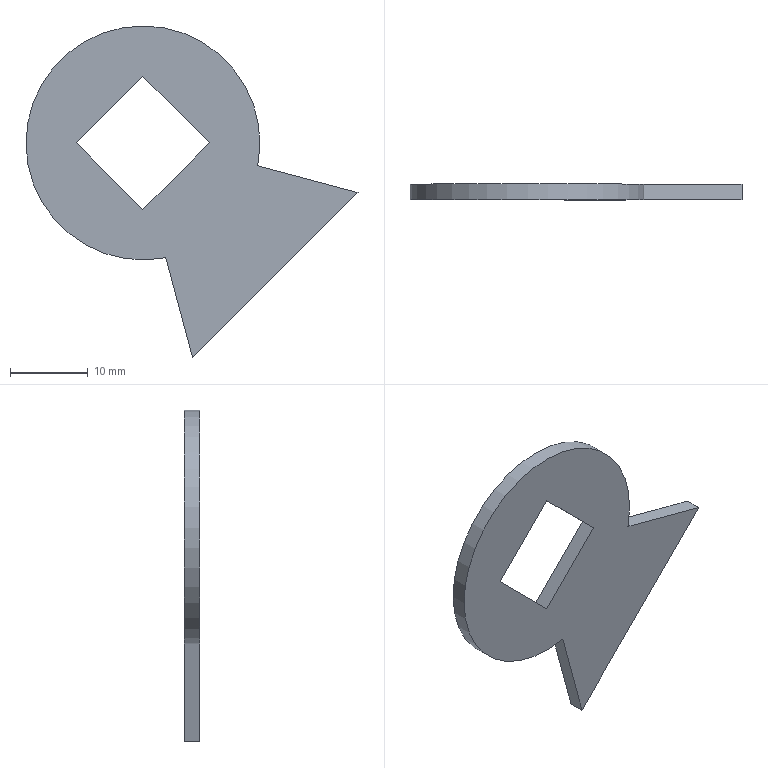Component | NX | LIMIT_PLATE | 1 solid | 10 faces | box 42.58 x 2 x 42.58 mm | volume 1607 mm3 | plane 9 | cylinder 1 | commonest cylinder face diameters 30 x1
STEP:
#1=CARTESIAN_POINT('',(0.,0.,0.));
#2=DIRECTION('',(0.,0.,1.));
#3=DIRECTION('',(1.,0.,0.));
#4=AXIS2_PLACEMENT_3D('',#1,#2,#3);
#5=CARTESIAN_POINT('',(-0.,-95.,-35.485));
#6=VERTEX_POINT('',#5);
#7=CARTESIAN_POINT('',(-8.485,-95.,-27.));
#8=VERTEX_POINT('',#7);
#9=CARTESIAN_POINT('',(-0.,-95.,-35.485));
#10=DIRECTION('',(-0.7071,0.,0.7071));
#11=VECTOR('',#10,1.);
#12=LINE('',#9,#11);
#13=CARTESIAN_POINT('',(-0.,-97.,-35.485));
#14=DIRECTION('',(-0.7071,0.,-0.7071));
#15=DIRECTION('',(0.7071,0.,-0.7071));
#16=AXIS2_PLACEMENT_3D('',#13,#14,#15);
#17=PLANE('',#16);
#18=CARTESIAN_POINT('',(0.,-2.));
#19=DIRECTION('',(-1.,0.));
#20=VECTOR('',#19,1.);
#21=LINE('',#18,#20);
#22=(GEOMETRIC_REPRESENTATION_CONTEXT(2)PARAMETRIC_REPRESENTATION_CONTEXT()REPRESENTATION_CONTEXT('',''));
#23=DEFINITIONAL_REPRESENTATION('',(#21),#22);
#24=PCURVE('',#17,#23);
#25=CARTESIAN_POINT('',(0.,-95.,-27.));
#26=DIRECTION('',(0.,1.,0.));
#27=DIRECTION('',(-0.7071,0.,-0.7071));
#28=AXIS2_PLACEMENT_3D('',#25,#26,#27);
#29=PLANE('',#28);
#30=CARTESIAN_POINT('',(6.,-6.));
#31=DIRECTION('',(0.,1.));
#32=VECTOR('',#31,1.);
#33=LINE('',#30,#32);
#34=(GEOMETRIC_REPRESENTATION_CONTEXT(2)PARAMETRIC_REPRESENTATION_CONTEXT()REPRESENTATION_CONTEXT('',''));
#35=DEFINITIONAL_REPRESENTATION('',(#33),#34);
#36=PCURVE('',#29,#35);
#37=SURFACE_CURVE('',#12,(#24,#36),.PCURVE_S1.);
#38=EDGE_CURVE('',#6,#8,#37,.T.);
#39=ORIENTED_EDGE('',*,*,#38,.T.);
#40=CARTESIAN_POINT('',(-8.485,-97.,-27.));
#41=VERTEX_POINT('',#40);
#42=CARTESIAN_POINT('',(-8.485,-97.,-27.));
#43=DIRECTION('',(0.,1.,0.));
#44=VECTOR('',#43,1.);
#45=LINE('',#42,#44);
#46=CARTESIAN_POINT('',(-12.,0.));
#47=DIRECTION('',(0.,-1.));
#48=VECTOR('',#47,1.);
#49=LINE('',#46,#48);
#50=(GEOMETRIC_REPRESENTATION_CONTEXT(2)PARAMETRIC_REPRESENTATION_CONTEXT()REPRESENTATION_CONTEXT('',''));
#51=DEFINITIONAL_REPRESENTATION('',(#49),#50);
#52=PCURVE('',#17,#51);
#53=CARTESIAN_POINT('',(-8.485,-97.,-27.));
#54=DIRECTION('',(-0.7071,0.,0.7071));
#55=DIRECTION('',(-0.7071,0.,-0.7071));
#56=AXIS2_PLACEMENT_3D('',#53,#54,#55);
#57=PLANE('',#56);
#58=CARTESIAN_POINT('',(0.,0.));
#59=DIRECTION('',(0.,-1.));
#60=VECTOR('',#59,1.);
#61=LINE('',#58,#60);
#62=(GEOMETRIC_REPRESENTATION_CONTEXT(2)PARAMETRIC_REPRESENTATION_CONTEXT()REPRESENTATION_CONTEXT('',''));
#63=DEFINITIONAL_REPRESENTATION('',(#61),#62);
#64=PCURVE('',#57,#63);
#65=SURFACE_CURVE('',#45,(#52,#64),.PCURVE_S1.);
#66=EDGE_CURVE('',#41,#8,#65,.T.);
#67=ORIENTED_EDGE('',*,*,#66,.F.);
#68=CARTESIAN_POINT('',(-0.,-97.,-35.485));
#69=VERTEX_POINT('',#68);
#70=CARTESIAN_POINT('',(-0.,-97.,-35.485));
#71=DIRECTION('',(-0.7071,0.,0.7071));
#72=VECTOR('',#71,1.);
#73=LINE('',#70,#72);
#74=CARTESIAN_POINT('',(0.,0.));
#75=DIRECTION('',(-1.,0.));
#76=VECTOR('',#75,1.);
#77=LINE('',#74,#76);
#78=(GEOMETRIC_REPRESENTATION_CONTEXT(2)PARAMETRIC_REPRESENTATION_CONTEXT()REPRESENTATION_CONTEXT('',''));
#79=DEFINITIONAL_REPRESENTATION('',(#77),#78);
#80=PCURVE('',#17,#79);
#81=CARTESIAN_POINT('',(0.,-97.,-27.));
#82=DIRECTION('',(0.,1.,0.));
#83=DIRECTION('',(-0.7071,0.,-0.7071));
#84=AXIS2_PLACEMENT_3D('',#81,#82,#83);
#85=PLANE('',#84);
#86=CARTESIAN_POINT('',(6.,-6.));
#87=DIRECTION('',(0.,1.));
#88=VECTOR('',#87,1.);
#89=LINE('',#86,#88);
#90=(GEOMETRIC_REPRESENTATION_CONTEXT(2)PARAMETRIC_REPRESENTATION_CONTEXT()REPRESENTATION_CONTEXT('',''));
#91=DEFINITIONAL_REPRESENTATION('',(#89),#90);
#92=PCURVE('',#85,#91);
#93=SURFACE_CURVE('',#73,(#80,#92),.PCURVE_S1.);
#94=EDGE_CURVE('',#69,#41,#93,.T.);
#95=ORIENTED_EDGE('',*,*,#94,.F.);
#96=CARTESIAN_POINT('',(-0.,-97.,-35.485));
#97=DIRECTION('',(0.,1.,0.));
#98=VECTOR('',#97,1.);
#99=LINE('',#96,#98);
#100=CARTESIAN_POINT('',(0.,0.));
#101=DIRECTION('',(0.,-1.));
#102=VECTOR('',#101,1.);
#103=LINE('',#100,#102);
#104=(GEOMETRIC_REPRESENTATION_CONTEXT(2)PARAMETRIC_REPRESENTATION_CONTEXT()REPRESENTATION_CONTEXT('',''));
#105=DEFINITIONAL_REPRESENTATION('',(#103),#104);
#106=PCURVE('',#17,#105);
#107=CARTESIAN_POINT('',(8.485,-97.,-27.));
#108=DIRECTION('',(0.7071,0.,-0.7071));
#109=DIRECTION('',(0.7071,0.,0.7071));
#110=AXIS2_PLACEMENT_3D('',#107,#108,#109);
#111=PLANE('',#110);
#112=CARTESIAN_POINT('',(-12.,0.));
#113=DIRECTION('',(0.,-1.));
#114=VECTOR('',#113,1.);
#115=LINE('',#112,#114);
#116=(GEOMETRIC_REPRESENTATION_CONTEXT(2)PARAMETRIC_REPRESENTATION_CONTEXT()REPRESENTATION_CONTEXT('',''));
#117=DEFINITIONAL_REPRESENTATION('',(#115),#116);
#118=PCURVE('',#111,#117);
#119=SURFACE_CURVE('',#99,(#106,#118),.PCURVE_S1.);
#120=EDGE_CURVE('',#69,#6,#119,.T.);
#121=ORIENTED_EDGE('',*,*,#120,.T.);
#122=EDGE_LOOP('',(#39,#67,#95,#121));
#123=FACE_BOUND('',#122,.T.);
#124=ADVANCED_FACE('',(#123),#17,.F.);
#125=CARTESIAN_POINT('',(8.485,-95.,-27.));
#126=VERTEX_POINT('',#125);
#127=CARTESIAN_POINT('',(8.485,-95.,-27.));
#128=DIRECTION('',(-0.7071,0.,-0.7071));
#129=VECTOR('',#128,1.);
#130=LINE('',#127,#129);
#131=CARTESIAN_POINT('',(0.,-2.));
#132=DIRECTION('',(-1.,0.));
#133=VECTOR('',#132,1.);
#134=LINE('',#131,#133);
#135=(GEOMETRIC_REPRESENTATION_CONTEXT(2)PARAMETRIC_REPRESENTATION_CONTEXT()REPRESENTATION_CONTEXT('',''));
#136=DEFINITIONAL_REPRESENTATION('',(#134),#135);
#137=PCURVE('',#111,#136);
#138=CARTESIAN_POINT('',(-6.,-6.));
#139=DIRECTION('',(1.,0.));
#140=VECTOR('',#139,1.);
#141=LINE('',#138,#140);
#142=(GEOMETRIC_REPRESENTATION_CONTEXT(2)PARAMETRIC_REPRESENTATION_CONTEXT()REPRESENTATION_CONTEXT('',''));
#143=DEFINITIONAL_REPRESENTATION('',(#141),#142);
#144=PCURVE('',#29,#143);
#145=SURFACE_CURVE('',#130,(#137,#144),.PCURVE_S1.);
#146=EDGE_CURVE('',#126,#6,#145,.T.);
#147=ORIENTED_EDGE('',*,*,#146,.T.);
#148=ORIENTED_EDGE('',*,*,#120,.F.);
#149=CARTESIAN_POINT('',(8.485,-97.,-27.));
#150=VERTEX_POINT('',#149);
#151=CARTESIAN_POINT('',(8.485,-97.,-27.));
#152=DIRECTION('',(-0.7071,0.,-0.7071));
#153=VECTOR('',#152,1.);
#154=LINE('',#151,#153);
#155=CARTESIAN_POINT('',(0.,0.));
#156=DIRECTION('',(-1.,0.));
#157=VECTOR('',#156,1.);
#158=LINE('',#155,#157);
#159=(GEOMETRIC_REPRESENTATION_CONTEXT(2)PARAMETRIC_REPRESENTATION_CONTEXT()REPRESENTATION_CONTEXT('',''));
#160=DEFINITIONAL_REPRESENTATION('',(#158),#159);
#161=PCURVE('',#111,#160);
#162=CARTESIAN_POINT('',(-6.,-6.));
#163=DIRECTION('',(1.,0.));
#164=VECTOR('',#163,1.);
#165=LINE('',#162,#164);
#166=(GEOMETRIC_REPRESENTATION_CONTEXT(2)PARAMETRIC_REPRESENTATION_CONTEXT()REPRESENTATION_CONTEXT('',''));
#167=DEFINITIONAL_REPRESENTATION('',(#165),#166);
#168=PCURVE('',#85,#167);
#169=SURFACE_CURVE('',#154,(#161,#168),.PCURVE_S1.);
#170=EDGE_CURVE('',#150,#69,#169,.T.);
#171=ORIENTED_EDGE('',*,*,#170,.F.);
#172=CARTESIAN_POINT('',(8.485,-97.,-27.));
#173=DIRECTION('',(0.,1.,0.));
#174=VECTOR('',#173,1.);
#175=LINE('',#172,#174);
#176=CARTESIAN_POINT('',(0.,0.));
#177=DIRECTION('',(0.,-1.));
#178=VECTOR('',#177,1.);
#179=LINE('',#176,#178);
#180=(GEOMETRIC_REPRESENTATION_CONTEXT(2)PARAMETRIC_REPRESENTATION_CONTEXT()REPRESENTATION_CONTEXT('',''));
#181=DEFINITIONAL_REPRESENTATION('',(#179),#180);
#182=PCURVE('',#111,#181);
#183=CARTESIAN_POINT('',(0.,-97.,-18.515));
#184=DIRECTION('',(0.7071,0.,0.7071));
#185=DIRECTION('',(-0.7071,0.,0.7071));
#186=AXIS2_PLACEMENT_3D('',#183,#184,#185);
#187=PLANE('',#186);
#188=CARTESIAN_POINT('',(-12.,0.));
#189=DIRECTION('',(0.,-1.));
#190=VECTOR('',#189,1.);
#191=LINE('',#188,#190);
#192=(GEOMETRIC_REPRESENTATION_CONTEXT(2)PARAMETRIC_REPRESENTATION_CONTEXT()REPRESENTATION_CONTEXT('',''));
#193=DEFINITIONAL_REPRESENTATION('',(#191),#192);
#194=PCURVE('',#187,#193);
#195=SURFACE_CURVE('',#175,(#182,#194),.PCURVE_S1.);
#196=EDGE_CURVE('',#150,#126,#195,.T.);
#197=ORIENTED_EDGE('',*,*,#196,.T.);
#198=EDGE_LOOP('',(#147,#148,#171,#197));
#199=FACE_BOUND('',#198,.T.);
#200=ADVANCED_FACE('',(#199),#111,.F.);
#201=CARTESIAN_POINT('',(0.,-95.,-18.515));
#202=VERTEX_POINT('',#201);
#203=CARTESIAN_POINT('',(0.,-95.,-18.515));
#204=DIRECTION('',(0.7071,0.,-0.7071));
#205=VECTOR('',#204,1.);
#206=LINE('',#203,#205);
#207=CARTESIAN_POINT('',(0.,-2.));
#208=DIRECTION('',(-1.,0.));
#209=VECTOR('',#208,1.);
#210=LINE('',#207,#209);
#211=(GEOMETRIC_REPRESENTATION_CONTEXT(2)PARAMETRIC_REPRESENTATION_CONTEXT()REPRESENTATION_CONTEXT('',''));
#212=DEFINITIONAL_REPRESENTATION('',(#210),#211);
#213=PCURVE('',#187,#212);
#214=CARTESIAN_POINT('',(-6.,6.));
#215=DIRECTION('',(0.,-1.));
#216=VECTOR('',#215,1.);
#217=LINE('',#214,#216);
#218=(GEOMETRIC_REPRESENTATION_CONTEXT(2)PARAMETRIC_REPRESENTATION_CONTEXT()REPRESENTATION_CONTEXT('',''));
#219=DEFINITIONAL_REPRESENTATION('',(#217),#218);
#220=PCURVE('',#29,#219);
#221=SURFACE_CURVE('',#206,(#213,#220),.PCURVE_S1.);
#222=EDGE_CURVE('',#202,#126,#221,.T.);
#223=ORIENTED_EDGE('',*,*,#222,.T.);
#224=ORIENTED_EDGE('',*,*,#196,.F.);
#225=CARTESIAN_POINT('',(0.,-97.,-18.515));
#226=VERTEX_POINT('',#225);
#227=CARTESIAN_POINT('',(0.,-97.,-18.515));
#228=DIRECTION('',(0.7071,0.,-0.7071));
#229=VECTOR('',#228,1.);
#230=LINE('',#227,#229);
#231=CARTESIAN_POINT('',(0.,0.));
#232=DIRECTION('',(-1.,0.));
#233=VECTOR('',#232,1.);
#234=LINE('',#231,#233);
#235=(GEOMETRIC_REPRESENTATION_CONTEXT(2)PARAMETRIC_REPRESENTATION_CONTEXT()REPRESENTATION_CONTEXT('',''));
#236=DEFINITIONAL_REPRESENTATION('',(#234),#235);
#237=PCURVE('',#187,#236);
#238=CARTESIAN_POINT('',(-6.,6.));
#239=DIRECTION('',(0.,-1.));
#240=VECTOR('',#239,1.);
#241=LINE('',#238,#240);
#242=(GEOMETRIC_REPRESENTATION_CONTEXT(2)PARAMETRIC_REPRESENTATION_CONTEXT()REPRESENTATION_CONTEXT('',''));
#243=DEFINITIONAL_REPRESENTATION('',(#241),#242);
#244=PCURVE('',#85,#243);
#245=SURFACE_CURVE('',#230,(#237,#244),.PCURVE_S1.);
#246=EDGE_CURVE('',#226,#150,#245,.T.);
#247=ORIENTED_EDGE('',*,*,#246,.F.);
#248=CARTESIAN_POINT('',(0.,-97.,-18.515));
#249=DIRECTION('',(0.,1.,0.));
#250=VECTOR('',#249,1.);
#251=LINE('',#248,#250);
#252=CARTESIAN_POINT('',(0.,0.));
#253=DIRECTION('',(0.,-1.));
#254=VECTOR('',#253,1.);
#255=LINE('',#252,#254);
#256=(GEOMETRIC_REPRESENTATION_CONTEXT(2)PARAMETRIC_REPRESENTATION_CONTEXT()REPRESENTATION_CONTEXT('',''));
#257=DEFINITIONAL_REPRESENTATION('',(#255),#256);
#258=PCURVE('',#187,#257);
#259=CARTESIAN_POINT('',(-12.,0.));
#260=DIRECTION('',(0.,-1.));
#261=VECTOR('',#260,1.);
#262=LINE('',#259,#261);
#263=(GEOMETRIC_REPRESENTATION_CONTEXT(2)PARAMETRIC_REPRESENTATION_CONTEXT()REPRESENTATION_CONTEXT('',''));
#264=DEFINITIONAL_REPRESENTATION('',(#262),#263);
#265=PCURVE('',#57,#264);
#266=SURFACE_CURVE('',#251,(#258,#265),.PCURVE_S1.);
#267=EDGE_CURVE('',#226,#202,#266,.T.);
#268=ORIENTED_EDGE('',*,*,#267,.T.);
#269=EDGE_LOOP('',(#223,#224,#247,#268));
#270=FACE_BOUND('',#269,.T.);
#271=ADVANCED_FACE('',(#270),#187,.F.);
#272=CARTESIAN_POINT('',(6.364,-95.,-54.577));
#273=VERTEX_POINT('',#272);
#274=CARTESIAN_POINT('',(2.917,-95.,-41.714));
#275=VERTEX_POINT('',#274);
#276=CARTESIAN_POINT('',(6.364,-95.,-54.577));
#277=DIRECTION('',(-0.2588,0.,0.9659));
#278=VECTOR('',#277,1.);
#279=LINE('',#276,#278);
#280=CARTESIAN_POINT('',(6.364,-97.,-54.577));
#281=DIRECTION('',(-0.9659,0.,-0.2588));
#282=DIRECTION('',(0.2588,0.,-0.9659));
#283=AXIS2_PLACEMENT_3D('',#280,#281,#282);
#284=PLANE('',#283);
#285=CARTESIAN_POINT('',(0.,-2.));
#286=DIRECTION('',(-1.,0.));
#287=VECTOR('',#286,1.);
#288=LINE('',#285,#287);
#289=(GEOMETRIC_REPRESENTATION_CONTEXT(2)PARAMETRIC_REPRESENTATION_CONTEXT()REPRESENTATION_CONTEXT('',''));
#290=DEFINITIONAL_REPRESENTATION('',(#288),#289);
#291=PCURVE('',#284,#290);
#292=CARTESIAN_POINT('',(15.,-24.));
#293=DIRECTION('',(-0.5,0.866));
#294=VECTOR('',#293,1.);
#295=LINE('',#292,#294);
#296=(GEOMETRIC_REPRESENTATION_CONTEXT(2)PARAMETRIC_REPRESENTATION_CONTEXT()REPRESENTATION_CONTEXT('',''));
#297=DEFINITIONAL_REPRESENTATION('',(#295),#296);
#298=PCURVE('',#29,#297);
#299=SURFACE_CURVE('',#279,(#291,#298),.PCURVE_S1.);
#300=EDGE_CURVE('',#273,#275,#299,.T.);
#301=ORIENTED_EDGE('',*,*,#300,.F.);
#302=CARTESIAN_POINT('',(6.364,-97.,-54.577));
#303=VERTEX_POINT('',#302);
#304=CARTESIAN_POINT('',(6.364,-97.,-54.577));
#305=DIRECTION('',(0.,1.,0.));
#306=VECTOR('',#305,1.);
#307=LINE('',#304,#306);
#308=CARTESIAN_POINT('',(0.,0.));
#309=DIRECTION('',(0.,-1.));
#310=VECTOR('',#309,1.);
#311=LINE('',#308,#310);
#312=(GEOMETRIC_REPRESENTATION_CONTEXT(2)PARAMETRIC_REPRESENTATION_CONTEXT()REPRESENTATION_CONTEXT('',''));
#313=DEFINITIONAL_REPRESENTATION('',(#311),#312);
#314=PCURVE('',#284,#313);
#315=CARTESIAN_POINT('',(16.971,-97.,-43.971));
#316=DIRECTION('',(0.7071,0.,-0.7071));
#317=DIRECTION('',(0.,1.,0.));
#318=AXIS2_PLACEMENT_3D('',#315,#316,#317);
#319=PLANE('',#318);
#320=CARTESIAN_POINT('',(0.,-15.));
#321=DIRECTION('',(1.,0.));
#322=VECTOR('',#321,1.);
#323=LINE('',#320,#322);
#324=(GEOMETRIC_REPRESENTATION_CONTEXT(2)PARAMETRIC_REPRESENTATION_CONTEXT()REPRESENTATION_CONTEXT('',''));
#325=DEFINITIONAL_REPRESENTATION('',(#323),#324);
#326=PCURVE('',#319,#325);
#327=SURFACE_CURVE('',#307,(#314,#326),.PCURVE_S1.);
#328=EDGE_CURVE('',#303,#273,#327,.T.);
#329=ORIENTED_EDGE('',*,*,#328,.F.);
#330=CARTESIAN_POINT('',(2.917,-97.,-41.714));
#331=VERTEX_POINT('',#330);
#332=CARTESIAN_POINT('',(6.364,-97.,-54.577));
#333=DIRECTION('',(-0.2588,0.,0.9659));
#334=VECTOR('',#333,1.);
#335=LINE('',#332,#334);
#336=CARTESIAN_POINT('',(0.,0.));
#337=DIRECTION('',(-1.,0.));
#338=VECTOR('',#337,1.);
#339=LINE('',#336,#338);
#340=(GEOMETRIC_REPRESENTATION_CONTEXT(2)PARAMETRIC_REPRESENTATION_CONTEXT()REPRESENTATION_CONTEXT('',''));
#341=DEFINITIONAL_REPRESENTATION('',(#339),#340);
#342=PCURVE('',#284,#341);
#343=CARTESIAN_POINT('',(15.,-24.));
#344=DIRECTION('',(-0.5,0.866));
#345=VECTOR('',#344,1.);
#346=LINE('',#343,#345);
#347=(GEOMETRIC_REPRESENTATION_CONTEXT(2)PARAMETRIC_REPRESENTATION_CONTEXT()REPRESENTATION_CONTEXT('',''));
#348=DEFINITIONAL_REPRESENTATION('',(#346),#347);
#349=PCURVE('',#85,#348);
#350=SURFACE_CURVE('',#335,(#342,#349),.PCURVE_S1.);
#351=EDGE_CURVE('',#303,#331,#350,.T.);
#352=ORIENTED_EDGE('',*,*,#351,.T.);
#353=CARTESIAN_POINT('',(2.917,-97.,-41.714));
#354=DIRECTION('',(0.,1.,0.));
#355=VECTOR('',#354,1.);
#356=LINE('',#353,#355);
#357=CARTESIAN_POINT('',(-13.317,0.));
#358=DIRECTION('',(0.,-1.));
#359=VECTOR('',#358,1.);
#360=LINE('',#357,#359);
#361=(GEOMETRIC_REPRESENTATION_CONTEXT(2)PARAMETRIC_REPRESENTATION_CONTEXT()REPRESENTATION_CONTEXT('',''));
#362=DEFINITIONAL_REPRESENTATION('',(#360),#361);
#363=PCURVE('',#284,#362);
#364=CARTESIAN_POINT('',(0.,-97.,-27.));
#365=DIRECTION('',(0.,1.,0.));
#366=DIRECTION('',(-0.7071,0.,-0.7071));
#367=AXIS2_PLACEMENT_3D('',#364,#365,#366);
#368=CYLINDRICAL_SURFACE('',#367,15.);
#369=CARTESIAN_POINT('',(-0.9811,0.));
#370=DIRECTION('',(0.,1.));
#371=VECTOR('',#370,1.);
#372=LINE('',#369,#371);
#373=(GEOMETRIC_REPRESENTATION_CONTEXT(2)PARAMETRIC_REPRESENTATION_CONTEXT()REPRESENTATION_CONTEXT('',''));
#374=DEFINITIONAL_REPRESENTATION('',(#372),#373);
#375=PCURVE('',#368,#374);
#376=SURFACE_CURVE('',#356,(#363,#375),.PCURVE_S1.);
#377=EDGE_CURVE('',#331,#275,#376,.T.);
#378=ORIENTED_EDGE('',*,*,#377,.T.);
#379=EDGE_LOOP('',(#301,#329,#352,#378));
#380=FACE_BOUND('',#379,.T.);
#381=ADVANCED_FACE('',(#380),#284,.T.);
#382=CARTESIAN_POINT('',(14.714,-95.,-29.917));
#383=VERTEX_POINT('',#382);
#384=CARTESIAN_POINT('',(0.,-95.,-27.));
#385=DIRECTION('',(0.,1.,0.));
#386=DIRECTION('',(0.7071,0.,0.7071));
#387=AXIS2_PLACEMENT_3D('',#384,#385,#386);
#388=CIRCLE('',#387,15.);
#389=CARTESIAN_POINT('',(-3.142,2.));
#390=DIRECTION('',(1.,0.));
#391=VECTOR('',#390,1.);
#392=LINE('',#389,#391);
#393=(GEOMETRIC_REPRESENTATION_CONTEXT(2)PARAMETRIC_REPRESENTATION_CONTEXT()REPRESENTATION_CONTEXT('',''));
#394=DEFINITIONAL_REPRESENTATION('',(#392),#393);
#395=PCURVE('',#368,#394);
#396=CARTESIAN_POINT('',(0.,0.));
#397=DIRECTION('',(-1.,0.));
#398=AXIS2_PLACEMENT_2D('',#396,#397);
#399=CIRCLE('',#398,15.);
#400=(GEOMETRIC_REPRESENTATION_CONTEXT(2)PARAMETRIC_REPRESENTATION_CONTEXT()REPRESENTATION_CONTEXT('',''));
#401=DEFINITIONAL_REPRESENTATION('',(#399),#400);
#402=PCURVE('',#29,#401);
#403=SURFACE_CURVE('',#388,(#395,#402),.PCURVE_S1.);
#404=EDGE_CURVE('',#275,#383,#403,.T.);
#405=ORIENTED_EDGE('',*,*,#404,.F.);
#406=ORIENTED_EDGE('',*,*,#377,.F.);
#407=CARTESIAN_POINT('',(14.714,-97.,-29.917));
#408=VERTEX_POINT('',#407);
#409=CARTESIAN_POINT('',(0.,-97.,-27.));
#410=DIRECTION('',(0.,1.,0.));
#411=DIRECTION('',(0.7071,0.,0.7071));
#412=AXIS2_PLACEMENT_3D('',#409,#410,#411);
#413=CIRCLE('',#412,15.);
#414=CARTESIAN_POINT('',(-3.142,0.));
#415=DIRECTION('',(1.,0.));
#416=VECTOR('',#415,1.);
#417=LINE('',#414,#416);
#418=(GEOMETRIC_REPRESENTATION_CONTEXT(2)PARAMETRIC_REPRESENTATION_CONTEXT()REPRESENTATION_CONTEXT('',''));
#419=DEFINITIONAL_REPRESENTATION('',(#417),#418);
#420=PCURVE('',#368,#419);
#421=CARTESIAN_POINT('',(0.,0.));
#422=DIRECTION('',(-1.,0.));
#423=AXIS2_PLACEMENT_2D('',#421,#422);
#424=CIRCLE('',#423,15.);
#425=(GEOMETRIC_REPRESENTATION_CONTEXT(2)PARAMETRIC_REPRESENTATION_CONTEXT()REPRESENTATION_CONTEXT('',''));
#426=DEFINITIONAL_REPRESENTATION('',(#424),#425);
#427=PCURVE('',#85,#426);
#428=SURFACE_CURVE('',#413,(#420,#427),.PCURVE_S1.);
#429=EDGE_CURVE('',#331,#408,#428,.T.);
#430=ORIENTED_EDGE('',*,*,#429,.T.);
#431=CARTESIAN_POINT('',(14.714,-97.,-29.917));
#432=DIRECTION('',(0.,1.,0.));
#433=VECTOR('',#432,1.);
#434=LINE('',#431,#433);
#435=CARTESIAN_POINT('',(4.123,0.));
#436=DIRECTION('',(0.,1.));
#437=VECTOR('',#436,1.);
#438=LINE('',#435,#437);
#439=(GEOMETRIC_REPRESENTATION_CONTEXT(2)PARAMETRIC_REPRESENTATION_CONTEXT()REPRESENTATION_CONTEXT('',''));
#440=DEFINITIONAL_REPRESENTATION('',(#438),#439);
#441=PCURVE('',#368,#440);
#442=CARTESIAN_POINT('',(14.714,-97.,-29.917));
#443=DIRECTION('',(0.2588,0.,0.9659));
#444=DIRECTION('',(-0.9659,0.,0.2588));
#445=AXIS2_PLACEMENT_3D('',#442,#443,#444);
#446=PLANE('',#445);
#447=CARTESIAN_POINT('',(0.,0.));
#448=DIRECTION('',(0.,-1.));
#449=VECTOR('',#448,1.);
#450=LINE('',#447,#449);
#451=(GEOMETRIC_REPRESENTATION_CONTEXT(2)PARAMETRIC_REPRESENTATION_CONTEXT()REPRESENTATION_CONTEXT('',''));
#452=DEFINITIONAL_REPRESENTATION('',(#450),#451);
#453=PCURVE('',#446,#452);
#454=SURFACE_CURVE('',#434,(#441,#453),.PCURVE_S1.);
#455=EDGE_CURVE('',#408,#383,#454,.T.);
#456=ORIENTED_EDGE('',*,*,#455,.T.);
#457=EDGE_LOOP('',(#405,#406,#430,#456));
#458=FACE_BOUND('',#457,.T.);
#459=ADVANCED_FACE('',(#458),#368,.T.);
#460=CARTESIAN_POINT('',(27.577,-95.,-33.364));
#461=VERTEX_POINT('',#460);
#462=CARTESIAN_POINT('',(14.714,-95.,-29.917));
#463=DIRECTION('',(0.9659,0.,-0.2588));
#464=VECTOR('',#463,1.);
#465=LINE('',#462,#464);
#466=CARTESIAN_POINT('',(0.,-2.));
#467=DIRECTION('',(-1.,0.));
#468=VECTOR('',#467,1.);
#469=LINE('',#466,#468);
#470=(GEOMETRIC_REPRESENTATION_CONTEXT(2)PARAMETRIC_REPRESENTATION_CONTEXT()REPRESENTATION_CONTEXT('',''));
#471=DEFINITIONAL_REPRESENTATION('',(#469),#470);
#472=PCURVE('',#446,#471);
#473=CARTESIAN_POINT('',(-8.341,-12.467));
#474=DIRECTION('',(-0.5,-0.866));
#475=VECTOR('',#474,1.);
#476=LINE('',#473,#475);
#477=(GEOMETRIC_REPRESENTATION_CONTEXT(2)PARAMETRIC_REPRESENTATION_CONTEXT()REPRESENTATION_CONTEXT('',''));
#478=DEFINITIONAL_REPRESENTATION('',(#476),#477);
#479=PCURVE('',#29,#478);
#480=SURFACE_CURVE('',#465,(#472,#479),.PCURVE_S1.);
#481=EDGE_CURVE('',#383,#461,#480,.T.);
#482=ORIENTED_EDGE('',*,*,#481,.F.);
#483=ORIENTED_EDGE('',*,*,#455,.F.);
#484=CARTESIAN_POINT('',(27.577,-97.,-33.364));
#485=VERTEX_POINT('',#484);
#486=CARTESIAN_POINT('',(14.714,-97.,-29.917));
#487=DIRECTION('',(0.9659,0.,-0.2588));
#488=VECTOR('',#487,1.);
#489=LINE('',#486,#488);
#490=CARTESIAN_POINT('',(0.,0.));
#491=DIRECTION('',(-1.,0.));
#492=VECTOR('',#491,1.);
#493=LINE('',#490,#492);
#494=(GEOMETRIC_REPRESENTATION_CONTEXT(2)PARAMETRIC_REPRESENTATION_CONTEXT()REPRESENTATION_CONTEXT('',''));
#495=DEFINITIONAL_REPRESENTATION('',(#493),#494);
#496=PCURVE('',#446,#495);
#497=CARTESIAN_POINT('',(-8.341,-12.467));
#498=DIRECTION('',(-0.5,-0.866));
#499=VECTOR('',#498,1.);
#500=LINE('',#497,#499);
#501=(GEOMETRIC_REPRESENTATION_CONTEXT(2)PARAMETRIC_REPRESENTATION_CONTEXT()REPRESENTATION_CONTEXT('',''));
#502=DEFINITIONAL_REPRESENTATION('',(#500),#501);
#503=PCURVE('',#85,#502);
#504=SURFACE_CURVE('',#489,(#496,#503),.PCURVE_S1.);
#505=EDGE_CURVE('',#408,#485,#504,.T.);
#506=ORIENTED_EDGE('',*,*,#505,.T.);
#507=CARTESIAN_POINT('',(27.577,-97.,-33.364));
#508=DIRECTION('',(0.,1.,0.));
#509=VECTOR('',#508,1.);
#510=LINE('',#507,#509);
#511=CARTESIAN_POINT('',(-13.317,0.));
#512=DIRECTION('',(0.,-1.));
#513=VECTOR('',#512,1.);
#514=LINE('',#511,#513);
#515=(GEOMETRIC_REPRESENTATION_CONTEXT(2)PARAMETRIC_REPRESENTATION_CONTEXT()REPRESENTATION_CONTEXT('',''));
#516=DEFINITIONAL_REPRESENTATION('',(#514),#515);
#517=PCURVE('',#446,#516);
#518=CARTESIAN_POINT('',(0.,15.));
#519=DIRECTION('',(1.,0.));
#520=VECTOR('',#519,1.);
#521=LINE('',#518,#520);
#522=(GEOMETRIC_REPRESENTATION_CONTEXT(2)PARAMETRIC_REPRESENTATION_CONTEXT()REPRESENTATION_CONTEXT('',''));
#523=DEFINITIONAL_REPRESENTATION('',(#521),#522);
#524=PCURVE('',#319,#523);
#525=SURFACE_CURVE('',#510,(#517,#524),.PCURVE_S1.);
#526=EDGE_CURVE('',#485,#461,#525,.T.);
#527=ORIENTED_EDGE('',*,*,#526,.T.);
#528=EDGE_LOOP('',(#482,#483,#506,#527));
#529=FACE_BOUND('',#528,.T.);
#530=ADVANCED_FACE('',(#529),#446,.T.);
#531=CARTESIAN_POINT('',(16.971,-95.,-43.971));
#532=DIRECTION('',(-0.7071,0.,-0.7071));
#533=VECTOR('',#532,1.);
#534=LINE('',#531,#533);
#535=CARTESIAN_POINT('',(2.,0.));
#536=DIRECTION('',(0.,-1.));
#537=VECTOR('',#536,1.);
#538=LINE('',#535,#537);
#539=(GEOMETRIC_REPRESENTATION_CONTEXT(2)PARAMETRIC_REPRESENTATION_CONTEXT()REPRESENTATION_CONTEXT('',''));
#540=DEFINITIONAL_REPRESENTATION('',(#538),#539);
#541=PCURVE('',#319,#540);
#542=CARTESIAN_POINT('',(0.,-24.));
#543=DIRECTION('',(1.,0.));
#544=VECTOR('',#543,1.);
#545=LINE('',#542,#544);
#546=(GEOMETRIC_REPRESENTATION_CONTEXT(2)PARAMETRIC_REPRESENTATION_CONTEXT()REPRESENTATION_CONTEXT('',''));
#547=DEFINITIONAL_REPRESENTATION('',(#545),#546);
#548=PCURVE('',#29,#547);
#549=SURFACE_CURVE('',#534,(#541,#548),.PCURVE_S1.);
#550=EDGE_CURVE('',#461,#273,#549,.T.);
#551=ORIENTED_EDGE('',*,*,#550,.F.);
#552=ORIENTED_EDGE('',*,*,#526,.F.);
#553=CARTESIAN_POINT('',(27.577,-97.,-33.364));
#554=DIRECTION('',(-0.7071,0.,-0.7071));
#555=VECTOR('',#554,1.);
#556=LINE('',#553,#555);
#557=CARTESIAN_POINT('',(0.,15.));
#558=DIRECTION('',(0.,-1.));
#559=VECTOR('',#558,1.);
#560=LINE('',#557,#559);
#561=(GEOMETRIC_REPRESENTATION_CONTEXT(2)PARAMETRIC_REPRESENTATION_CONTEXT()REPRESENTATION_CONTEXT('',''));
#562=DEFINITIONAL_REPRESENTATION('',(#560),#561);
#563=PCURVE('',#319,#562);
#564=CARTESIAN_POINT('',(-15.,-24.));
#565=DIRECTION('',(1.,0.));
#566=VECTOR('',#565,1.);
#567=LINE('',#564,#566);
#568=(GEOMETRIC_REPRESENTATION_CONTEXT(2)PARAMETRIC_REPRESENTATION_CONTEXT()REPRESENTATION_CONTEXT('',''));
#569=DEFINITIONAL_REPRESENTATION('',(#567),#568);
#570=PCURVE('',#85,#569);
#571=SURFACE_CURVE('',#556,(#563,#570),.PCURVE_S1.);
#572=EDGE_CURVE('',#485,#303,#571,.T.);
#573=ORIENTED_EDGE('',*,*,#572,.T.);
#574=ORIENTED_EDGE('',*,*,#328,.T.);
#575=EDGE_LOOP('',(#551,#552,#573,#574));
#576=FACE_BOUND('',#575,.T.);
#577=ADVANCED_FACE('',(#576),#319,.T.);
#578=CARTESIAN_POINT('',(-8.485,-95.,-27.));
#579=DIRECTION('',(0.7071,0.,0.7071));
#580=VECTOR('',#579,1.);
#581=LINE('',#578,#580);
#582=CARTESIAN_POINT('',(0.,-2.));
#583=DIRECTION('',(-1.,0.));
#584=VECTOR('',#583,1.);
#585=LINE('',#582,#584);
#586=(GEOMETRIC_REPRESENTATION_CONTEXT(2)PARAMETRIC_REPRESENTATION_CONTEXT()REPRESENTATION_CONTEXT('',''));
#587=DEFINITIONAL_REPRESENTATION('',(#585),#586);
#588=PCURVE('',#57,#587);
#589=CARTESIAN_POINT('',(6.,6.));
#590=DIRECTION('',(-1.,0.));
#591=VECTOR('',#590,1.);
#592=LINE('',#589,#591);
#593=(GEOMETRIC_REPRESENTATION_CONTEXT(2)PARAMETRIC_REPRESENTATION_CONTEXT()REPRESENTATION_CONTEXT('',''));
#594=DEFINITIONAL_REPRESENTATION('',(#592),#593);
#595=PCURVE('',#29,#594);
#596=SURFACE_CURVE('',#581,(#588,#595),.PCURVE_S1.);
#597=EDGE_CURVE('',#8,#202,#596,.T.);
#598=ORIENTED_EDGE('',*,*,#597,.T.);
#599=ORIENTED_EDGE('',*,*,#267,.F.);
#600=CARTESIAN_POINT('',(-8.485,-97.,-27.));
#601=DIRECTION('',(0.7071,0.,0.7071));
#602=VECTOR('',#601,1.);
#603=LINE('',#600,#602);
#604=CARTESIAN_POINT('',(0.,0.));
#605=DIRECTION('',(-1.,0.));
#606=VECTOR('',#605,1.);
#607=LINE('',#604,#606);
#608=(GEOMETRIC_REPRESENTATION_CONTEXT(2)PARAMETRIC_REPRESENTATION_CONTEXT()REPRESENTATION_CONTEXT('',''));
#609=DEFINITIONAL_REPRESENTATION('',(#607),#608);
#610=PCURVE('',#57,#609);
#611=CARTESIAN_POINT('',(6.,6.));
#612=DIRECTION('',(-1.,0.));
#613=VECTOR('',#612,1.);
#614=LINE('',#611,#613);
#615=(GEOMETRIC_REPRESENTATION_CONTEXT(2)PARAMETRIC_REPRESENTATION_CONTEXT()REPRESENTATION_CONTEXT('',''));
#616=DEFINITIONAL_REPRESENTATION('',(#614),#615);
#617=PCURVE('',#85,#616);
#618=SURFACE_CURVE('',#603,(#610,#617),.PCURVE_S1.);
#619=EDGE_CURVE('',#41,#226,#618,.T.);
#620=ORIENTED_EDGE('',*,*,#619,.F.);
#621=ORIENTED_EDGE('',*,*,#66,.T.);
#622=EDGE_LOOP('',(#598,#599,#620,#621));
#623=FACE_BOUND('',#622,.T.);
#624=ADVANCED_FACE('',(#623),#57,.F.);
#625=ORIENTED_EDGE('',*,*,#351,.F.);
#626=ORIENTED_EDGE('',*,*,#572,.F.);
#627=ORIENTED_EDGE('',*,*,#505,.F.);
#628=ORIENTED_EDGE('',*,*,#429,.F.);
#629=EDGE_LOOP('',(#625,#626,#627,#628));
#630=FACE_BOUND('',#629,.T.);
#631=ORIENTED_EDGE('',*,*,#94,.T.);
#632=ORIENTED_EDGE('',*,*,#619,.T.);
#633=ORIENTED_EDGE('',*,*,#246,.T.);
#634=ORIENTED_EDGE('',*,*,#170,.T.);
#635=EDGE_LOOP('',(#631,#632,#633,#634));
#636=FACE_BOUND('',#635,.T.);
#637=ADVANCED_FACE('',(#630,#636),#85,.F.);
#638=ORIENTED_EDGE('',*,*,#300,.T.);
#639=ORIENTED_EDGE('',*,*,#404,.T.);
#640=ORIENTED_EDGE('',*,*,#481,.T.);
#641=ORIENTED_EDGE('',*,*,#550,.T.);
#642=EDGE_LOOP('',(#638,#639,#640,#641));
#643=FACE_BOUND('',#642,.T.);
#644=ORIENTED_EDGE('',*,*,#38,.F.);
#645=ORIENTED_EDGE('',*,*,#146,.F.);
#646=ORIENTED_EDGE('',*,*,#222,.F.);
#647=ORIENTED_EDGE('',*,*,#597,.F.);
#648=EDGE_LOOP('',(#644,#645,#646,#647));
#649=FACE_BOUND('',#648,.T.);
#650=ADVANCED_FACE('',(#643,#649),#29,.T.);
#651=CLOSED_SHELL('',(#124,#200,#271,#381,#459,#530,#577,#624,#637,#650));
#652=MANIFOLD_SOLID_BREP('',#651);
#653=(LENGTH_UNIT()NAMED_UNIT(*)SI_UNIT(.MILLI.,.METRE.));
#654=UNCERTAINTY_MEASURE_WITH_UNIT(LENGTH_MEASURE(0.0000001),#653,'','');
#655=(NAMED_UNIT(*)PLANE_ANGLE_UNIT()SI_UNIT($,.RADIAN.));
#656=(NAMED_UNIT(*)SI_UNIT($,.STERADIAN.)SOLID_ANGLE_UNIT());
#657=(GEOMETRIC_REPRESENTATION_CONTEXT(3)GLOBAL_UNCERTAINTY_ASSIGNED_CONTEXT((#654))GLOBAL_UNIT_ASSIGNED_CONTEXT((#653,#655,#656))REPRESENTATION_CONTEXT('',''));
#658=ADVANCED_BREP_SHAPE_REPRESENTATION('',(#4,#652),#657);